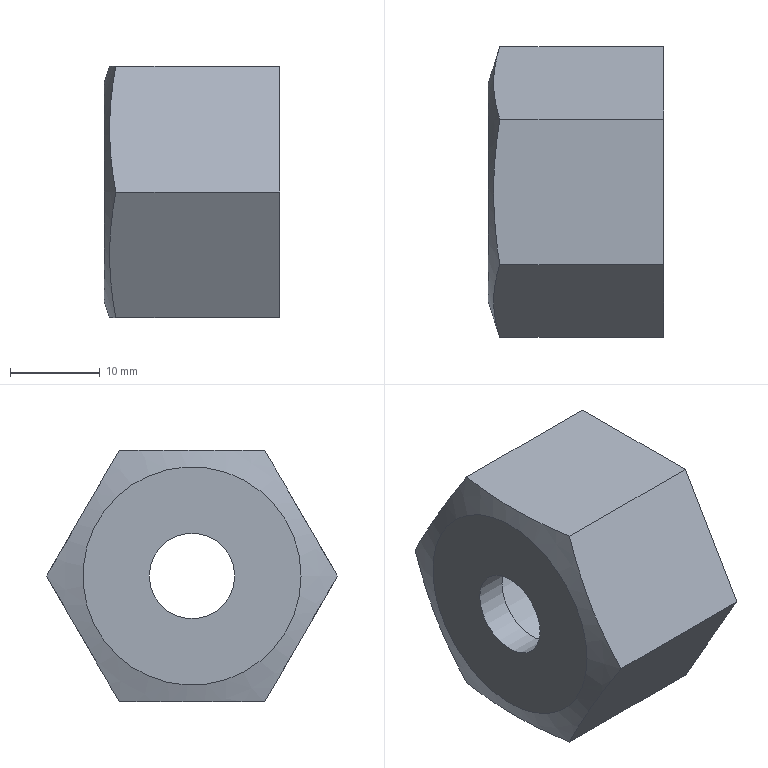Component | NX | LARGE_NUT | 1 solid | 12 faces | box 19.5 x 32.33 x 28 mm | volume 5656 mm3 | plane 9 | cylinder 2 | cone 1 | commonest cylinder face diameters 24 x1 9.5 x1
STEP:
#1=CARTESIAN_POINT('',(0.,0.,0.));
#2=DIRECTION('',(0.,0.,1.));
#3=DIRECTION('',(1.,0.,0.));
#4=AXIS2_PLACEMENT_3D('',#1,#2,#3);
#5=CARTESIAN_POINT('',(-168.222,-8.083,269.5));
#6=VERTEX_POINT('',#5);
#7=CARTESIAN_POINT('',(-150.,-8.083,269.5));
#8=VERTEX_POINT('',#7);
#9=CARTESIAN_POINT('',(-169.5,-8.083,269.5));
#10=DIRECTION('',(1.,0.,0.));
#11=VECTOR('',#10,1.);
#12=LINE('',#9,#11);
#13=CARTESIAN_POINT('',(-169.5,-16.166,255.5));
#14=DIRECTION('',(0.,0.866,-0.5));
#15=DIRECTION('',(0.,-0.5,-0.866));
#16=AXIS2_PLACEMENT_3D('',#13,#14,#15);
#17=PLANE('',#16);
#18=CARTESIAN_POINT('',(-16.166,0.));
#19=DIRECTION('',(0.,-1.));
#20=VECTOR('',#19,1.);
#21=LINE('',#18,#20);
#22=(GEOMETRIC_REPRESENTATION_CONTEXT(2)PARAMETRIC_REPRESENTATION_CONTEXT()REPRESENTATION_CONTEXT('',''));
#23=DEFINITIONAL_REPRESENTATION('',(#21),#22);
#24=PCURVE('',#17,#23);
#25=CARTESIAN_POINT('',(-169.5,-8.083,269.5));
#26=DIRECTION('',(0.,0.,-1.));
#27=DIRECTION('',(0.,-1.,-0.));
#28=AXIS2_PLACEMENT_3D('',#25,#26,#27);
#29=PLANE('',#28);
#30=CARTESIAN_POINT('',(0.,0.));
#31=DIRECTION('',(0.,-1.));
#32=VECTOR('',#31,1.);
#33=LINE('',#30,#32);
#34=(GEOMETRIC_REPRESENTATION_CONTEXT(2)PARAMETRIC_REPRESENTATION_CONTEXT()REPRESENTATION_CONTEXT('',''));
#35=DEFINITIONAL_REPRESENTATION('',(#33),#34);
#36=PCURVE('',#29,#35);
#37=SURFACE_CURVE('',#12,(#24,#36),.PCURVE_S1.);
#38=EDGE_CURVE('',#6,#8,#37,.T.);
#39=ORIENTED_EDGE('',*,*,#38,.F.);
#40=CARTESIAN_POINT('',(-168.222,-16.166,255.5));
#41=VERTEX_POINT('',#40);
#42=CARTESIAN_POINT('',(-168.222,-8.083,269.5));
#43=CARTESIAN_POINT('',(-168.648,-9.43,267.167));
#44=CARTESIAN_POINT('',(-169.166,-12.124,262.5));
#45=CARTESIAN_POINT('',(-168.648,-14.819,257.833));
#46=CARTESIAN_POINT('',(-168.222,-16.166,255.5));
#47=B_SPLINE_CURVE_WITH_KNOTS('',3,(#42,#43,#44,#45,#46),.UNSPECIFIED.,.F.,.F.,(4,1,4),(0.,0.5,1.),.QUASI_UNIFORM_KNOTS.);
#48=CARTESIAN_POINT('',(-16.166,-1.278));
#49=CARTESIAN_POINT('',(-13.472,-0.8519));
#50=CARTESIAN_POINT('',(-8.083,-0.3342));
#51=CARTESIAN_POINT('',(-2.694,-0.8519));
#52=CARTESIAN_POINT('',(0.,-1.278));
#53=B_SPLINE_CURVE_WITH_KNOTS('',3,(#48,#49,#50,#51,#52),.UNSPECIFIED.,.F.,.F.,(4,1,4),(0.,0.5,1.),.QUASI_UNIFORM_KNOTS.);
#54=(GEOMETRIC_REPRESENTATION_CONTEXT(2)PARAMETRIC_REPRESENTATION_CONTEXT()REPRESENTATION_CONTEXT('',''));
#55=DEFINITIONAL_REPRESENTATION('',(#53),#54);
#56=PCURVE('',#17,#55);
#57=CARTESIAN_POINT('',(-169.5,-0.,255.5));
#58=DIRECTION('',(1.,0.,0.));
#59=DIRECTION('',(0.,-1.,0.));
#60=AXIS2_PLACEMENT_3D('',#57,#58,#59);
#61=CONICAL_SURFACE('',#60,12.124,1.265);
#62=CARTESIAN_POINT('',(5.236,1.278));
#63=CARTESIAN_POINT('',(5.249,1.239));
#64=CARTESIAN_POINT('',(5.276,1.164));
#65=CARTESIAN_POINT('',(5.318,1.061));
#66=CARTESIAN_POINT('',(5.362,0.966));
#67=CARTESIAN_POINT('',(5.407,0.8809));
#68=CARTESIAN_POINT('',(5.454,0.8058));
#69=CARTESIAN_POINT('',(5.503,0.7413));
#70=CARTESIAN_POINT('',(5.552,0.6878));
#71=CARTESIAN_POINT('',(5.603,0.6458));
#72=CARTESIAN_POINT('',(5.655,0.6155));
#73=CARTESIAN_POINT('',(5.707,0.5972));
#74=CARTESIAN_POINT('',(5.76,0.591));
#75=CARTESIAN_POINT('',(5.812,0.5972));
#76=CARTESIAN_POINT('',(5.864,0.6155));
#77=CARTESIAN_POINT('',(5.916,0.6458));
#78=CARTESIAN_POINT('',(5.967,0.6878));
#79=CARTESIAN_POINT('',(6.016,0.7413));
#80=CARTESIAN_POINT('',(6.065,0.8058));
#81=CARTESIAN_POINT('',(6.112,0.8809));
#82=CARTESIAN_POINT('',(6.157,0.966));
#83=CARTESIAN_POINT('',(6.201,1.061));
#84=CARTESIAN_POINT('',(6.243,1.164));
#85=CARTESIAN_POINT('',(6.27,1.239));
#86=CARTESIAN_POINT('',(6.283,1.278));
#87=B_SPLINE_CURVE_WITH_KNOTS('',3,(#62,#63,#64,#65,#66,#67,#68,#69,#70,#71,#72,#73,#74,#75,#76,#77,#78,#79,#80,#81,#82,#83,#84,#85,#86),.UNSPECIFIED.,.F.,.F.,(4,1,1,1,1,1,1,1,1,1,1,1,1,1,1,1,1,1,1,1,1,1,4),(0.,0.04545,0.09091,0.1364,0.1818,0.2273,0.2727,0.3182,0.3636,0.4091,0.4545,0.5,0.5455,0.5909,0.6364,0.6818,0.7273,0.7727,0.8182,0.8636,0.9091,0.9545,1.),.QUASI_UNIFORM_KNOTS.);
#88=(GEOMETRIC_REPRESENTATION_CONTEXT(2)PARAMETRIC_REPRESENTATION_CONTEXT()REPRESENTATION_CONTEXT('',''));
#89=DEFINITIONAL_REPRESENTATION('',(#87),#88);
#90=PCURVE('',#61,#89);
#91=SURFACE_CURVE('',#47,(#56,#90),.PCURVE_S1.);
#92=EDGE_CURVE('',#6,#41,#91,.T.);
#93=ORIENTED_EDGE('',*,*,#92,.T.);
#94=CARTESIAN_POINT('',(-150.,-16.166,255.5));
#95=VERTEX_POINT('',#94);
#96=CARTESIAN_POINT('',(-169.5,-16.166,255.5));
#97=DIRECTION('',(1.,0.,0.));
#98=VECTOR('',#97,1.);
#99=LINE('',#96,#98);
#100=CARTESIAN_POINT('',(0.,0.));
#101=DIRECTION('',(0.,-1.));
#102=VECTOR('',#101,1.);
#103=LINE('',#100,#102);
#104=(GEOMETRIC_REPRESENTATION_CONTEXT(2)PARAMETRIC_REPRESENTATION_CONTEXT()REPRESENTATION_CONTEXT('',''));
#105=DEFINITIONAL_REPRESENTATION('',(#103),#104);
#106=PCURVE('',#17,#105);
#107=CARTESIAN_POINT('',(-169.5,-8.083,241.5));
#108=DIRECTION('',(0.,0.866,0.5));
#109=DIRECTION('',(0.,0.5,-0.866));
#110=AXIS2_PLACEMENT_3D('',#107,#108,#109);
#111=PLANE('',#110);
#112=CARTESIAN_POINT('',(-16.166,0.));
#113=DIRECTION('',(0.,-1.));
#114=VECTOR('',#113,1.);
#115=LINE('',#112,#114);
#116=(GEOMETRIC_REPRESENTATION_CONTEXT(2)PARAMETRIC_REPRESENTATION_CONTEXT()REPRESENTATION_CONTEXT('',''));
#117=DEFINITIONAL_REPRESENTATION('',(#115),#116);
#118=PCURVE('',#111,#117);
#119=SURFACE_CURVE('',#99,(#106,#118),.PCURVE_S1.);
#120=EDGE_CURVE('',#41,#95,#119,.T.);
#121=ORIENTED_EDGE('',*,*,#120,.T.);
#122=CARTESIAN_POINT('',(-150.,-16.166,255.5));
#123=DIRECTION('',(0.,0.5,0.866));
#124=VECTOR('',#123,1.);
#125=LINE('',#122,#124);
#126=CARTESIAN_POINT('',(0.,-19.5));
#127=DIRECTION('',(-1.,0.));
#128=VECTOR('',#127,1.);
#129=LINE('',#126,#128);
#130=(GEOMETRIC_REPRESENTATION_CONTEXT(2)PARAMETRIC_REPRESENTATION_CONTEXT()REPRESENTATION_CONTEXT('',''));
#131=DEFINITIONAL_REPRESENTATION('',(#129),#130);
#132=PCURVE('',#17,#131);
#133=CARTESIAN_POINT('',(-150.,-0.,255.5));
#134=DIRECTION('',(-1.,0.,0.));
#135=DIRECTION('',(0.,1.,0.));
#136=AXIS2_PLACEMENT_3D('',#133,#134,#135);
#137=PLANE('',#136);
#138=CARTESIAN_POINT('',(-16.166,0.));
#139=DIRECTION('',(0.5,-0.866));
#140=VECTOR('',#139,1.);
#141=LINE('',#138,#140);
#142=(GEOMETRIC_REPRESENTATION_CONTEXT(2)PARAMETRIC_REPRESENTATION_CONTEXT()REPRESENTATION_CONTEXT('',''));
#143=DEFINITIONAL_REPRESENTATION('',(#141),#142);
#144=PCURVE('',#137,#143);
#145=SURFACE_CURVE('',#125,(#132,#144),.PCURVE_S1.);
#146=EDGE_CURVE('',#95,#8,#145,.T.);
#147=ORIENTED_EDGE('',*,*,#146,.T.);
#148=EDGE_LOOP('',(#39,#93,#121,#147));
#149=FACE_BOUND('',#148,.T.);
#150=ADVANCED_FACE('',(#149),#17,.F.);
#151=CARTESIAN_POINT('',(-168.222,8.083,269.5));
#152=VERTEX_POINT('',#151);
#153=CARTESIAN_POINT('',(-150.,8.083,269.5));
#154=VERTEX_POINT('',#153);
#155=CARTESIAN_POINT('',(-169.5,8.083,269.5));
#156=DIRECTION('',(1.,0.,0.));
#157=VECTOR('',#156,1.);
#158=LINE('',#155,#157);
#159=CARTESIAN_POINT('',(-16.166,0.));
#160=DIRECTION('',(0.,-1.));
#161=VECTOR('',#160,1.);
#162=LINE('',#159,#161);
#163=(GEOMETRIC_REPRESENTATION_CONTEXT(2)PARAMETRIC_REPRESENTATION_CONTEXT()REPRESENTATION_CONTEXT('',''));
#164=DEFINITIONAL_REPRESENTATION('',(#162),#163);
#165=PCURVE('',#29,#164);
#166=CARTESIAN_POINT('',(-169.5,8.083,269.5));
#167=DIRECTION('',(0.,-0.866,-0.5));
#168=DIRECTION('',(0.,-0.5,0.866));
#169=AXIS2_PLACEMENT_3D('',#166,#167,#168);
#170=PLANE('',#169);
#171=CARTESIAN_POINT('',(0.,0.));
#172=DIRECTION('',(0.,-1.));
#173=VECTOR('',#172,1.);
#174=LINE('',#171,#173);
#175=(GEOMETRIC_REPRESENTATION_CONTEXT(2)PARAMETRIC_REPRESENTATION_CONTEXT()REPRESENTATION_CONTEXT('',''));
#176=DEFINITIONAL_REPRESENTATION('',(#174),#175);
#177=PCURVE('',#170,#176);
#178=SURFACE_CURVE('',#158,(#165,#177),.PCURVE_S1.);
#179=EDGE_CURVE('',#152,#154,#178,.T.);
#180=ORIENTED_EDGE('',*,*,#179,.F.);
#181=CARTESIAN_POINT('',(-168.222,8.083,269.5));
#182=CARTESIAN_POINT('',(-168.646,5.403,269.5));
#183=CARTESIAN_POINT('',(-168.906,2.717,269.5));
#184=CARTESIAN_POINT('',(-168.908,-2.675,269.5));
#185=CARTESIAN_POINT('',(-168.647,-5.393,269.5));
#186=CARTESIAN_POINT('',(-168.222,-8.083,269.5));
#187=B_SPLINE_CURVE_WITH_KNOTS('',3,(#181,#182,#183,#184,#185,#186),.UNSPECIFIED.,.F.,.F.,(4,2,4),(0.,0.5,1.),.UNSPECIFIED.);
#188=CARTESIAN_POINT('',(-16.166,-1.278));
#189=CARTESIAN_POINT('',(-13.486,-0.8542));
#190=CARTESIAN_POINT('',(-10.799,-0.5944));
#191=CARTESIAN_POINT('',(-5.408,-0.5918));
#192=CARTESIAN_POINT('',(-2.69,-0.8527));
#193=CARTESIAN_POINT('',(0.,-1.278));
#194=B_SPLINE_CURVE_WITH_KNOTS('',3,(#188,#189,#190,#191,#192,#193),.UNSPECIFIED.,.F.,.F.,(4,2,4),(0.,0.5,1.),.UNSPECIFIED.);
#195=(GEOMETRIC_REPRESENTATION_CONTEXT(2)PARAMETRIC_REPRESENTATION_CONTEXT()REPRESENTATION_CONTEXT('',''));
#196=DEFINITIONAL_REPRESENTATION('',(#194),#195);
#197=PCURVE('',#29,#196);
#198=CARTESIAN_POINT('',(4.189,1.278));
#199=CARTESIAN_POINT('',(4.202,1.239));
#200=CARTESIAN_POINT('',(4.229,1.165));
#201=CARTESIAN_POINT('',(4.27,1.062));
#202=CARTESIAN_POINT('',(4.314,0.9673));
#203=CARTESIAN_POINT('',(4.359,0.8823));
#204=CARTESIAN_POINT('',(4.406,0.8073));
#205=CARTESIAN_POINT('',(4.454,0.7427));
#206=CARTESIAN_POINT('',(4.504,0.6891));
#207=CARTESIAN_POINT('',(4.555,0.6468));
#208=CARTESIAN_POINT('',(4.606,0.6162));
#209=CARTESIAN_POINT('',(4.658,0.5975));
#210=CARTESIAN_POINT('',(4.711,0.591));
#211=CARTESIAN_POINT('',(4.763,0.5968));
#212=CARTESIAN_POINT('',(4.816,0.6149));
#213=CARTESIAN_POINT('',(4.868,0.645));
#214=CARTESIAN_POINT('',(4.919,0.687));
#215=CARTESIAN_POINT('',(4.969,0.7406));
#216=CARTESIAN_POINT('',(5.017,0.8052));
#217=CARTESIAN_POINT('',(5.065,0.8805));
#218=CARTESIAN_POINT('',(5.11,0.9658));
#219=CARTESIAN_POINT('',(5.154,1.061));
#220=CARTESIAN_POINT('',(5.196,1.165));
#221=CARTESIAN_POINT('',(5.223,1.239));
#222=CARTESIAN_POINT('',(5.236,1.278));
#223=B_SPLINE_CURVE_WITH_KNOTS('',3,(#198,#199,#200,#201,#202,#203,#204,#205,#206,#207,#208,#209,#210,#211,#212,#213,#214,#215,#216,#217,#218,#219,#220,#221,#222),.UNSPECIFIED.,.F.,.F.,(4,1,1,1,1,1,1,1,1,1,1,1,1,1,1,1,1,1,1,1,1,1,4),(0.,0.04545,0.09091,0.1364,0.1818,0.2273,0.2727,0.3182,0.3636,0.4091,0.4545,0.5,0.5455,0.5909,0.6364,0.6818,0.7273,0.7727,0.8182,0.8636,0.9091,0.9545,1.),.QUASI_UNIFORM_KNOTS.);
#224=(GEOMETRIC_REPRESENTATION_CONTEXT(2)PARAMETRIC_REPRESENTATION_CONTEXT()REPRESENTATION_CONTEXT('',''));
#225=DEFINITIONAL_REPRESENTATION('',(#223),#224);
#226=PCURVE('',#61,#225);
#227=SURFACE_CURVE('',#187,(#197,#226),.PCURVE_S1.);
#228=EDGE_CURVE('',#152,#6,#227,.T.);
#229=ORIENTED_EDGE('',*,*,#228,.T.);
#230=ORIENTED_EDGE('',*,*,#38,.T.);
#231=CARTESIAN_POINT('',(-150.,-8.083,269.5));
#232=DIRECTION('',(0.,1.,0.));
#233=VECTOR('',#232,1.);
#234=LINE('',#231,#233);
#235=CARTESIAN_POINT('',(0.,-19.5));
#236=DIRECTION('',(-1.,0.));
#237=VECTOR('',#236,1.);
#238=LINE('',#235,#237);
#239=(GEOMETRIC_REPRESENTATION_CONTEXT(2)PARAMETRIC_REPRESENTATION_CONTEXT()REPRESENTATION_CONTEXT('',''));
#240=DEFINITIONAL_REPRESENTATION('',(#238),#239);
#241=PCURVE('',#29,#240);
#242=CARTESIAN_POINT('',(-8.083,-14.));
#243=DIRECTION('',(1.,-0.));
#244=VECTOR('',#243,1.);
#245=LINE('',#242,#244);
#246=(GEOMETRIC_REPRESENTATION_CONTEXT(2)PARAMETRIC_REPRESENTATION_CONTEXT()REPRESENTATION_CONTEXT('',''));
#247=DEFINITIONAL_REPRESENTATION('',(#245),#246);
#248=PCURVE('',#137,#247);
#249=SURFACE_CURVE('',#234,(#241,#248),.PCURVE_S1.);
#250=EDGE_CURVE('',#8,#154,#249,.T.);
#251=ORIENTED_EDGE('',*,*,#250,.T.);
#252=EDGE_LOOP('',(#180,#229,#230,#251));
#253=FACE_BOUND('',#252,.T.);
#254=ADVANCED_FACE('',(#253),#29,.F.);
#255=CARTESIAN_POINT('',(-168.222,16.166,255.5));
#256=VERTEX_POINT('',#255);
#257=CARTESIAN_POINT('',(-150.,16.166,255.5));
#258=VERTEX_POINT('',#257);
#259=CARTESIAN_POINT('',(-169.5,16.166,255.5));
#260=DIRECTION('',(1.,0.,0.));
#261=VECTOR('',#260,1.);
#262=LINE('',#259,#261);
#263=CARTESIAN_POINT('',(-16.166,0.));
#264=DIRECTION('',(0.,-1.));
#265=VECTOR('',#264,1.);
#266=LINE('',#263,#265);
#267=(GEOMETRIC_REPRESENTATION_CONTEXT(2)PARAMETRIC_REPRESENTATION_CONTEXT()REPRESENTATION_CONTEXT('',''));
#268=DEFINITIONAL_REPRESENTATION('',(#266),#267);
#269=PCURVE('',#170,#268);
#270=CARTESIAN_POINT('',(-169.5,16.166,255.5));
#271=DIRECTION('',(0.,-0.866,0.5));
#272=DIRECTION('',(0.,0.5,0.866));
#273=AXIS2_PLACEMENT_3D('',#270,#271,#272);
#274=PLANE('',#273);
#275=CARTESIAN_POINT('',(0.,0.));
#276=DIRECTION('',(0.,-1.));
#277=VECTOR('',#276,1.);
#278=LINE('',#275,#277);
#279=(GEOMETRIC_REPRESENTATION_CONTEXT(2)PARAMETRIC_REPRESENTATION_CONTEXT()REPRESENTATION_CONTEXT('',''));
#280=DEFINITIONAL_REPRESENTATION('',(#278),#279);
#281=PCURVE('',#274,#280);
#282=SURFACE_CURVE('',#262,(#269,#281),.PCURVE_S1.);
#283=EDGE_CURVE('',#256,#258,#282,.T.);
#284=ORIENTED_EDGE('',*,*,#283,.F.);
#285=CARTESIAN_POINT('',(-168.222,16.166,255.5));
#286=CARTESIAN_POINT('',(-168.648,14.819,257.833));
#287=CARTESIAN_POINT('',(-169.166,12.124,262.5));
#288=CARTESIAN_POINT('',(-168.648,9.43,267.167));
#289=CARTESIAN_POINT('',(-168.222,8.083,269.5));
#290=B_SPLINE_CURVE_WITH_KNOTS('',3,(#285,#286,#287,#288,#289),.UNSPECIFIED.,.F.,.F.,(4,1,4),(0.,0.5,1.),.QUASI_UNIFORM_KNOTS.);
#291=CARTESIAN_POINT('',(-16.166,-1.278));
#292=CARTESIAN_POINT('',(-13.472,-0.8519));
#293=CARTESIAN_POINT('',(-8.083,-0.3342));
#294=CARTESIAN_POINT('',(-2.694,-0.8519));
#295=CARTESIAN_POINT('',(0.,-1.278));
#296=B_SPLINE_CURVE_WITH_KNOTS('',3,(#291,#292,#293,#294,#295),.UNSPECIFIED.,.F.,.F.,(4,1,4),(0.,0.5,1.),.QUASI_UNIFORM_KNOTS.);
#297=(GEOMETRIC_REPRESENTATION_CONTEXT(2)PARAMETRIC_REPRESENTATION_CONTEXT()REPRESENTATION_CONTEXT('',''));
#298=DEFINITIONAL_REPRESENTATION('',(#296),#297);
#299=PCURVE('',#170,#298);
#300=CARTESIAN_POINT('',(3.142,1.278));
#301=CARTESIAN_POINT('',(3.155,1.239));
#302=CARTESIAN_POINT('',(3.182,1.164));
#303=CARTESIAN_POINT('',(3.224,1.061));
#304=CARTESIAN_POINT('',(3.267,0.966));
#305=CARTESIAN_POINT('',(3.313,0.8809));
#306=CARTESIAN_POINT('',(3.36,0.8058));
#307=CARTESIAN_POINT('',(3.408,0.7413));
#308=CARTESIAN_POINT('',(3.458,0.6878));
#309=CARTESIAN_POINT('',(3.509,0.6458));
#310=CARTESIAN_POINT('',(3.561,0.6155));
#311=CARTESIAN_POINT('',(3.613,0.5972));
#312=CARTESIAN_POINT('',(3.665,0.591));
#313=CARTESIAN_POINT('',(3.718,0.5972));
#314=CARTESIAN_POINT('',(3.77,0.6155));
#315=CARTESIAN_POINT('',(3.822,0.6458));
#316=CARTESIAN_POINT('',(3.872,0.6878));
#317=CARTESIAN_POINT('',(3.922,0.7413));
#318=CARTESIAN_POINT('',(3.971,0.8058));
#319=CARTESIAN_POINT('',(4.018,0.8809));
#320=CARTESIAN_POINT('',(4.063,0.966));
#321=CARTESIAN_POINT('',(4.107,1.061));
#322=CARTESIAN_POINT('',(4.149,1.164));
#323=CARTESIAN_POINT('',(4.176,1.239));
#324=CARTESIAN_POINT('',(4.189,1.278));
#325=B_SPLINE_CURVE_WITH_KNOTS('',3,(#300,#301,#302,#303,#304,#305,#306,#307,#308,#309,#310,#311,#312,#313,#314,#315,#316,#317,#318,#319,#320,#321,#322,#323,#324),.UNSPECIFIED.,.F.,.F.,(4,1,1,1,1,1,1,1,1,1,1,1,1,1,1,1,1,1,1,1,1,1,4),(0.,0.04545,0.09091,0.1364,0.1818,0.2273,0.2727,0.3182,0.3636,0.4091,0.4545,0.5,0.5455,0.5909,0.6364,0.6818,0.7273,0.7727,0.8182,0.8636,0.9091,0.9545,1.),.QUASI_UNIFORM_KNOTS.);
#326=(GEOMETRIC_REPRESENTATION_CONTEXT(2)PARAMETRIC_REPRESENTATION_CONTEXT()REPRESENTATION_CONTEXT('',''));
#327=DEFINITIONAL_REPRESENTATION('',(#325),#326);
#328=PCURVE('',#61,#327);
#329=SURFACE_CURVE('',#290,(#299,#328),.PCURVE_S1.);
#330=EDGE_CURVE('',#256,#152,#329,.T.);
#331=ORIENTED_EDGE('',*,*,#330,.T.);
#332=ORIENTED_EDGE('',*,*,#179,.T.);
#333=CARTESIAN_POINT('',(-150.,8.083,269.5));
#334=DIRECTION('',(0.,0.5,-0.866));
#335=VECTOR('',#334,1.);
#336=LINE('',#333,#335);
#337=CARTESIAN_POINT('',(0.,-19.5));
#338=DIRECTION('',(-1.,0.));
#339=VECTOR('',#338,1.);
#340=LINE('',#337,#339);
#341=(GEOMETRIC_REPRESENTATION_CONTEXT(2)PARAMETRIC_REPRESENTATION_CONTEXT()REPRESENTATION_CONTEXT('',''));
#342=DEFINITIONAL_REPRESENTATION('',(#340),#341);
#343=PCURVE('',#170,#342);
#344=CARTESIAN_POINT('',(8.083,-14.));
#345=DIRECTION('',(0.5,0.866));
#346=VECTOR('',#345,1.);
#347=LINE('',#344,#346);
#348=(GEOMETRIC_REPRESENTATION_CONTEXT(2)PARAMETRIC_REPRESENTATION_CONTEXT()REPRESENTATION_CONTEXT('',''));
#349=DEFINITIONAL_REPRESENTATION('',(#347),#348);
#350=PCURVE('',#137,#349);
#351=SURFACE_CURVE('',#336,(#343,#350),.PCURVE_S1.);
#352=EDGE_CURVE('',#154,#258,#351,.T.);
#353=ORIENTED_EDGE('',*,*,#352,.T.);
#354=EDGE_LOOP('',(#284,#331,#332,#353));
#355=FACE_BOUND('',#354,.T.);
#356=ADVANCED_FACE('',(#355),#170,.F.);
#357=CARTESIAN_POINT('',(-168.222,8.083,241.5));
#358=VERTEX_POINT('',#357);
#359=CARTESIAN_POINT('',(-150.,8.083,241.5));
#360=VERTEX_POINT('',#359);
#361=CARTESIAN_POINT('',(-169.5,8.083,241.5));
#362=DIRECTION('',(1.,0.,0.));
#363=VECTOR('',#362,1.);
#364=LINE('',#361,#363);
#365=CARTESIAN_POINT('',(-16.166,0.));
#366=DIRECTION('',(0.,-1.));
#367=VECTOR('',#366,1.);
#368=LINE('',#365,#367);
#369=(GEOMETRIC_REPRESENTATION_CONTEXT(2)PARAMETRIC_REPRESENTATION_CONTEXT()REPRESENTATION_CONTEXT('',''));
#370=DEFINITIONAL_REPRESENTATION('',(#368),#369);
#371=PCURVE('',#274,#370);
#372=CARTESIAN_POINT('',(-169.5,8.083,241.5));
#373=DIRECTION('',(0.,-0.,1.));
#374=DIRECTION('',(0.,1.,0.));
#375=AXIS2_PLACEMENT_3D('',#372,#373,#374);
#376=PLANE('',#375);
#377=CARTESIAN_POINT('',(0.,0.));
#378=DIRECTION('',(0.,-1.));
#379=VECTOR('',#378,1.);
#380=LINE('',#377,#379);
#381=(GEOMETRIC_REPRESENTATION_CONTEXT(2)PARAMETRIC_REPRESENTATION_CONTEXT()REPRESENTATION_CONTEXT('',''));
#382=DEFINITIONAL_REPRESENTATION('',(#380),#381);
#383=PCURVE('',#376,#382);
#384=SURFACE_CURVE('',#364,(#371,#383),.PCURVE_S1.);
#385=EDGE_CURVE('',#358,#360,#384,.T.);
#386=ORIENTED_EDGE('',*,*,#385,.F.);
#387=CARTESIAN_POINT('',(-168.222,8.083,241.5));
#388=CARTESIAN_POINT('',(-168.648,9.43,243.833));
#389=CARTESIAN_POINT('',(-169.166,12.124,248.5));
#390=CARTESIAN_POINT('',(-168.648,14.819,253.167));
#391=CARTESIAN_POINT('',(-168.222,16.166,255.5));
#392=B_SPLINE_CURVE_WITH_KNOTS('',3,(#387,#388,#389,#390,#391),.UNSPECIFIED.,.F.,.F.,(4,1,4),(0.,0.5,1.),.UNSPECIFIED.);
#393=CARTESIAN_POINT('',(-16.166,-1.278));
#394=CARTESIAN_POINT('',(-13.472,-0.8519));
#395=CARTESIAN_POINT('',(-8.083,-0.3342));
#396=CARTESIAN_POINT('',(-2.694,-0.8519));
#397=CARTESIAN_POINT('',(0.,-1.278));
#398=B_SPLINE_CURVE_WITH_KNOTS('',3,(#393,#394,#395,#396,#397),.UNSPECIFIED.,.F.,.F.,(4,1,4),(0.,0.5,1.),.UNSPECIFIED.);
#399=(GEOMETRIC_REPRESENTATION_CONTEXT(2)PARAMETRIC_REPRESENTATION_CONTEXT()REPRESENTATION_CONTEXT('',''));
#400=DEFINITIONAL_REPRESENTATION('',(#398),#399);
#401=PCURVE('',#274,#400);
#402=CARTESIAN_POINT('',(2.094,1.278));
#403=CARTESIAN_POINT('',(2.108,1.239));
#404=CARTESIAN_POINT('',(2.134,1.164));
#405=CARTESIAN_POINT('',(2.176,1.061));
#406=CARTESIAN_POINT('',(2.22,0.966));
#407=CARTESIAN_POINT('',(2.266,0.8809));
#408=CARTESIAN_POINT('',(2.313,0.8058));
#409=CARTESIAN_POINT('',(2.361,0.7413));
#410=CARTESIAN_POINT('',(2.411,0.6878));
#411=CARTESIAN_POINT('',(2.462,0.6458));
#412=CARTESIAN_POINT('',(2.513,0.6155));
#413=CARTESIAN_POINT('',(2.566,0.5972));
#414=CARTESIAN_POINT('',(2.618,0.591));
#415=CARTESIAN_POINT('',(2.67,0.5972));
#416=CARTESIAN_POINT('',(2.723,0.6155));
#417=CARTESIAN_POINT('',(2.774,0.6458));
#418=CARTESIAN_POINT('',(2.825,0.6878));
#419=CARTESIAN_POINT('',(2.875,0.7413));
#420=CARTESIAN_POINT('',(2.923,0.8058));
#421=CARTESIAN_POINT('',(2.97,0.8809));
#422=CARTESIAN_POINT('',(3.016,0.966));
#423=CARTESIAN_POINT('',(3.06,1.061));
#424=CARTESIAN_POINT('',(3.102,1.164));
#425=CARTESIAN_POINT('',(3.128,1.239));
#426=CARTESIAN_POINT('',(3.142,1.278));
#427=B_SPLINE_CURVE_WITH_KNOTS('',3,(#402,#403,#404,#405,#406,#407,#408,#409,#410,#411,#412,#413,#414,#415,#416,#417,#418,#419,#420,#421,#422,#423,#424,#425,#426),.UNSPECIFIED.,.F.,.F.,(4,1,1,1,1,1,1,1,1,1,1,1,1,1,1,1,1,1,1,1,1,1,4),(0.,0.04545,0.09091,0.1364,0.1818,0.2273,0.2727,0.3182,0.3636,0.4091,0.4545,0.5,0.5455,0.5909,0.6364,0.6818,0.7273,0.7727,0.8182,0.8636,0.9091,0.9545,1.),.QUASI_UNIFORM_KNOTS.);
#428=(GEOMETRIC_REPRESENTATION_CONTEXT(2)PARAMETRIC_REPRESENTATION_CONTEXT()REPRESENTATION_CONTEXT('',''));
#429=DEFINITIONAL_REPRESENTATION('',(#427),#428);
#430=PCURVE('',#61,#429);
#431=SURFACE_CURVE('',#392,(#401,#430),.PCURVE_S1.);
#432=EDGE_CURVE('',#358,#256,#431,.T.);
#433=ORIENTED_EDGE('',*,*,#432,.T.);
#434=ORIENTED_EDGE('',*,*,#283,.T.);
#435=CARTESIAN_POINT('',(-150.,16.166,255.5));
#436=DIRECTION('',(0.,-0.5,-0.866));
#437=VECTOR('',#436,1.);
#438=LINE('',#435,#437);
#439=CARTESIAN_POINT('',(0.,-19.5));
#440=DIRECTION('',(-1.,0.));
#441=VECTOR('',#440,1.);
#442=LINE('',#439,#441);
#443=(GEOMETRIC_REPRESENTATION_CONTEXT(2)PARAMETRIC_REPRESENTATION_CONTEXT()REPRESENTATION_CONTEXT('',''));
#444=DEFINITIONAL_REPRESENTATION('',(#442),#443);
#445=PCURVE('',#274,#444);
#446=CARTESIAN_POINT('',(16.166,0.));
#447=DIRECTION('',(-0.5,0.866));
#448=VECTOR('',#447,1.);
#449=LINE('',#446,#448);
#450=(GEOMETRIC_REPRESENTATION_CONTEXT(2)PARAMETRIC_REPRESENTATION_CONTEXT()REPRESENTATION_CONTEXT('',''));
#451=DEFINITIONAL_REPRESENTATION('',(#449),#450);
#452=PCURVE('',#137,#451);
#453=SURFACE_CURVE('',#438,(#445,#452),.PCURVE_S1.);
#454=EDGE_CURVE('',#258,#360,#453,.T.);
#455=ORIENTED_EDGE('',*,*,#454,.T.);
#456=EDGE_LOOP('',(#386,#433,#434,#455));
#457=FACE_BOUND('',#456,.T.);
#458=ADVANCED_FACE('',(#457),#274,.F.);
#459=CARTESIAN_POINT('',(-168.222,-8.083,241.5));
#460=VERTEX_POINT('',#459);
#461=CARTESIAN_POINT('',(-150.,-8.083,241.5));
#462=VERTEX_POINT('',#461);
#463=CARTESIAN_POINT('',(-169.5,-8.083,241.5));
#464=DIRECTION('',(1.,0.,0.));
#465=VECTOR('',#464,1.);
#466=LINE('',#463,#465);
#467=CARTESIAN_POINT('',(-16.166,0.));
#468=DIRECTION('',(0.,-1.));
#469=VECTOR('',#468,1.);
#470=LINE('',#467,#469);
#471=(GEOMETRIC_REPRESENTATION_CONTEXT(2)PARAMETRIC_REPRESENTATION_CONTEXT()REPRESENTATION_CONTEXT('',''));
#472=DEFINITIONAL_REPRESENTATION('',(#470),#471);
#473=PCURVE('',#376,#472);
#474=CARTESIAN_POINT('',(0.,0.));
#475=DIRECTION('',(0.,-1.));
#476=VECTOR('',#475,1.);
#477=LINE('',#474,#476);
#478=(GEOMETRIC_REPRESENTATION_CONTEXT(2)PARAMETRIC_REPRESENTATION_CONTEXT()REPRESENTATION_CONTEXT('',''));
#479=DEFINITIONAL_REPRESENTATION('',(#477),#478);
#480=PCURVE('',#111,#479);
#481=SURFACE_CURVE('',#466,(#473,#480),.PCURVE_S1.);
#482=EDGE_CURVE('',#460,#462,#481,.T.);
#483=ORIENTED_EDGE('',*,*,#482,.F.);
#484=CARTESIAN_POINT('',(-168.222,-8.083,241.5));
#485=CARTESIAN_POINT('',(-168.647,-5.393,241.5));
#486=CARTESIAN_POINT('',(-168.908,-2.675,241.5));
#487=CARTESIAN_POINT('',(-168.906,2.717,241.5));
#488=CARTESIAN_POINT('',(-168.646,5.403,241.5));
#489=CARTESIAN_POINT('',(-168.222,8.083,241.5));
#490=B_SPLINE_CURVE_WITH_KNOTS('',3,(#484,#485,#486,#487,#488,#489),.UNSPECIFIED.,.F.,.F.,(4,2,4),(0.,0.5,1.),.UNSPECIFIED.);
#491=CARTESIAN_POINT('',(-16.166,-1.278));
#492=CARTESIAN_POINT('',(-13.476,-0.8527));
#493=CARTESIAN_POINT('',(-10.758,-0.5918));
#494=CARTESIAN_POINT('',(-5.366,-0.5944));
#495=CARTESIAN_POINT('',(-2.68,-0.8542));
#496=CARTESIAN_POINT('',(0.,-1.278));
#497=B_SPLINE_CURVE_WITH_KNOTS('',3,(#491,#492,#493,#494,#495,#496),.UNSPECIFIED.,.F.,.F.,(4,2,4),(0.,0.5,1.),.UNSPECIFIED.);
#498=(GEOMETRIC_REPRESENTATION_CONTEXT(2)PARAMETRIC_REPRESENTATION_CONTEXT()REPRESENTATION_CONTEXT('',''));
#499=DEFINITIONAL_REPRESENTATION('',(#497),#498);
#500=PCURVE('',#376,#499);
#501=CARTESIAN_POINT('',(1.047,1.278));
#502=CARTESIAN_POINT('',(1.06,1.239));
#503=CARTESIAN_POINT('',(1.087,1.165));
#504=CARTESIAN_POINT('',(1.129,1.061));
#505=CARTESIAN_POINT('',(1.173,0.9658));
#506=CARTESIAN_POINT('',(1.219,0.8805));
#507=CARTESIAN_POINT('',(1.266,0.8052));
#508=CARTESIAN_POINT('',(1.315,0.7406));
#509=CARTESIAN_POINT('',(1.365,0.687));
#510=CARTESIAN_POINT('',(1.416,0.645));
#511=CARTESIAN_POINT('',(1.467,0.6149));
#512=CARTESIAN_POINT('',(1.52,0.5968));
#513=CARTESIAN_POINT('',(1.572,0.591));
#514=CARTESIAN_POINT('',(1.625,0.5975));
#515=CARTESIAN_POINT('',(1.677,0.6162));
#516=CARTESIAN_POINT('',(1.729,0.6468));
#517=CARTESIAN_POINT('',(1.779,0.6891));
#518=CARTESIAN_POINT('',(1.829,0.7427));
#519=CARTESIAN_POINT('',(1.877,0.8073));
#520=CARTESIAN_POINT('',(1.924,0.8823));
#521=CARTESIAN_POINT('',(1.969,0.9673));
#522=CARTESIAN_POINT('',(2.013,1.062));
#523=CARTESIAN_POINT('',(2.055,1.165));
#524=CARTESIAN_POINT('',(2.081,1.239));
#525=CARTESIAN_POINT('',(2.094,1.278));
#526=B_SPLINE_CURVE_WITH_KNOTS('',3,(#501,#502,#503,#504,#505,#506,#507,#508,#509,#510,#511,#512,#513,#514,#515,#516,#517,#518,#519,#520,#521,#522,#523,#524,#525),.UNSPECIFIED.,.F.,.F.,(4,1,1,1,1,1,1,1,1,1,1,1,1,1,1,1,1,1,1,1,1,1,4),(0.,0.04545,0.09091,0.1364,0.1818,0.2273,0.2727,0.3182,0.3636,0.4091,0.4545,0.5,0.5455,0.5909,0.6364,0.6818,0.7273,0.7727,0.8182,0.8636,0.9091,0.9545,1.),.QUASI_UNIFORM_KNOTS.);
#527=(GEOMETRIC_REPRESENTATION_CONTEXT(2)PARAMETRIC_REPRESENTATION_CONTEXT()REPRESENTATION_CONTEXT('',''));
#528=DEFINITIONAL_REPRESENTATION('',(#526),#527);
#529=PCURVE('',#61,#528);
#530=SURFACE_CURVE('',#490,(#500,#529),.PCURVE_S1.);
#531=EDGE_CURVE('',#460,#358,#530,.T.);
#532=ORIENTED_EDGE('',*,*,#531,.T.);
#533=ORIENTED_EDGE('',*,*,#385,.T.);
#534=CARTESIAN_POINT('',(-150.,8.083,241.5));
#535=DIRECTION('',(0.,-1.,-0.));
#536=VECTOR('',#535,1.);
#537=LINE('',#534,#536);
#538=CARTESIAN_POINT('',(0.,-19.5));
#539=DIRECTION('',(-1.,0.));
#540=VECTOR('',#539,1.);
#541=LINE('',#538,#540);
#542=(GEOMETRIC_REPRESENTATION_CONTEXT(2)PARAMETRIC_REPRESENTATION_CONTEXT()REPRESENTATION_CONTEXT('',''));
#543=DEFINITIONAL_REPRESENTATION('',(#541),#542);
#544=PCURVE('',#376,#543);
#545=CARTESIAN_POINT('',(8.083,14.));
#546=DIRECTION('',(-1.,0.));
#547=VECTOR('',#546,1.);
#548=LINE('',#545,#547);
#549=(GEOMETRIC_REPRESENTATION_CONTEXT(2)PARAMETRIC_REPRESENTATION_CONTEXT()REPRESENTATION_CONTEXT('',''));
#550=DEFINITIONAL_REPRESENTATION('',(#548),#549);
#551=PCURVE('',#137,#550);
#552=SURFACE_CURVE('',#537,(#544,#551),.PCURVE_S1.);
#553=EDGE_CURVE('',#360,#462,#552,.T.);
#554=ORIENTED_EDGE('',*,*,#553,.T.);
#555=EDGE_LOOP('',(#483,#532,#533,#554));
#556=FACE_BOUND('',#555,.T.);
#557=ADVANCED_FACE('',(#556),#376,.F.);
#558=ORIENTED_EDGE('',*,*,#120,.F.);
#559=CARTESIAN_POINT('',(-168.222,-16.166,255.5));
#560=CARTESIAN_POINT('',(-168.648,-14.819,253.167));
#561=CARTESIAN_POINT('',(-169.166,-12.124,248.5));
#562=CARTESIAN_POINT('',(-168.648,-9.43,243.833));
#563=CARTESIAN_POINT('',(-168.222,-8.083,241.5));
#564=B_SPLINE_CURVE_WITH_KNOTS('',3,(#559,#560,#561,#562,#563),.UNSPECIFIED.,.F.,.F.,(4,1,4),(0.,0.5,1.),.UNSPECIFIED.);
#565=CARTESIAN_POINT('',(-16.166,-1.278));
#566=CARTESIAN_POINT('',(-13.472,-0.8519));
#567=CARTESIAN_POINT('',(-8.083,-0.3342));
#568=CARTESIAN_POINT('',(-2.694,-0.8519));
#569=CARTESIAN_POINT('',(0.,-1.278));
#570=B_SPLINE_CURVE_WITH_KNOTS('',3,(#565,#566,#567,#568,#569),.UNSPECIFIED.,.F.,.F.,(4,1,4),(0.,0.5,1.),.UNSPECIFIED.);
#571=(GEOMETRIC_REPRESENTATION_CONTEXT(2)PARAMETRIC_REPRESENTATION_CONTEXT()REPRESENTATION_CONTEXT('',''));
#572=DEFINITIONAL_REPRESENTATION('',(#570),#571);
#573=PCURVE('',#111,#572);
#574=CARTESIAN_POINT('',(0.,1.278));
#575=CARTESIAN_POINT('',(0.01312,1.239));
#576=CARTESIAN_POINT('',(0.03996,1.164));
#577=CARTESIAN_POINT('',(0.082,1.061));
#578=CARTESIAN_POINT('',(0.1258,0.966));
#579=CARTESIAN_POINT('',(0.1712,0.8809));
#580=CARTESIAN_POINT('',(0.2183,0.8058));
#581=CARTESIAN_POINT('',(0.2667,0.7413));
#582=CARTESIAN_POINT('',(0.3165,0.6878));
#583=CARTESIAN_POINT('',(0.3673,0.6458));
#584=CARTESIAN_POINT('',(0.4189,0.6155));
#585=CARTESIAN_POINT('',(0.4711,0.5972));
#586=CARTESIAN_POINT('',(0.5236,0.591));
#587=CARTESIAN_POINT('',(0.5761,0.5972));
#588=CARTESIAN_POINT('',(0.6283,0.6155));
#589=CARTESIAN_POINT('',(0.6799,0.6458));
#590=CARTESIAN_POINT('',(0.7307,0.6878));
#591=CARTESIAN_POINT('',(0.7805,0.7413));
#592=CARTESIAN_POINT('',(0.8289,0.8058));
#593=CARTESIAN_POINT('',(0.876,0.8809));
#594=CARTESIAN_POINT('',(0.9214,0.966));
#595=CARTESIAN_POINT('',(0.9652,1.061));
#596=CARTESIAN_POINT('',(1.007,1.164));
#597=CARTESIAN_POINT('',(1.034,1.239));
#598=CARTESIAN_POINT('',(1.047,1.278));
#599=B_SPLINE_CURVE_WITH_KNOTS('',3,(#574,#575,#576,#577,#578,#579,#580,#581,#582,#583,#584,#585,#586,#587,#588,#589,#590,#591,#592,#593,#594,#595,#596,#597,#598),.UNSPECIFIED.,.F.,.F.,(4,1,1,1,1,1,1,1,1,1,1,1,1,1,1,1,1,1,1,1,1,1,4),(0.,0.04545,0.09091,0.1364,0.1818,0.2273,0.2727,0.3182,0.3636,0.4091,0.4545,0.5,0.5455,0.5909,0.6364,0.6818,0.7273,0.7727,0.8182,0.8636,0.9091,0.9545,1.),.QUASI_UNIFORM_KNOTS.);
#600=(GEOMETRIC_REPRESENTATION_CONTEXT(2)PARAMETRIC_REPRESENTATION_CONTEXT()REPRESENTATION_CONTEXT('',''));
#601=DEFINITIONAL_REPRESENTATION('',(#599),#600);
#602=PCURVE('',#61,#601);
#603=SURFACE_CURVE('',#564,(#573,#602),.PCURVE_S1.);
#604=EDGE_CURVE('',#41,#460,#603,.T.);
#605=ORIENTED_EDGE('',*,*,#604,.T.);
#606=ORIENTED_EDGE('',*,*,#482,.T.);
#607=CARTESIAN_POINT('',(-150.,-8.083,241.5));
#608=DIRECTION('',(0.,-0.5,0.866));
#609=VECTOR('',#608,1.);
#610=LINE('',#607,#609);
#611=CARTESIAN_POINT('',(0.,-19.5));
#612=DIRECTION('',(-1.,0.));
#613=VECTOR('',#612,1.);
#614=LINE('',#611,#613);
#615=(GEOMETRIC_REPRESENTATION_CONTEXT(2)PARAMETRIC_REPRESENTATION_CONTEXT()REPRESENTATION_CONTEXT('',''));
#616=DEFINITIONAL_REPRESENTATION('',(#614),#615);
#617=PCURVE('',#111,#616);
#618=CARTESIAN_POINT('',(-8.083,14.));
#619=DIRECTION('',(-0.5,-0.866));
#620=VECTOR('',#619,1.);
#621=LINE('',#618,#620);
#622=(GEOMETRIC_REPRESENTATION_CONTEXT(2)PARAMETRIC_REPRESENTATION_CONTEXT()REPRESENTATION_CONTEXT('',''));
#623=DEFINITIONAL_REPRESENTATION('',(#621),#622);
#624=PCURVE('',#137,#623);
#625=SURFACE_CURVE('',#610,(#617,#624),.PCURVE_S1.);
#626=EDGE_CURVE('',#462,#95,#625,.T.);
#627=ORIENTED_EDGE('',*,*,#626,.T.);
#628=EDGE_LOOP('',(#558,#605,#606,#627));
#629=FACE_BOUND('',#628,.T.);
#630=ADVANCED_FACE('',(#629),#111,.F.);
#631=CARTESIAN_POINT('',(-150.,12.,255.5));
#632=VERTEX_POINT('',#631);
#633=CARTESIAN_POINT('',(-150.,-0.,255.5));
#634=DIRECTION('',(1.,0.,0.));
#635=DIRECTION('',(0.,1.,0.));
#636=AXIS2_PLACEMENT_3D('',#633,#634,#635);
#637=CIRCLE('',#636,12.);
#638=CARTESIAN_POINT('',(12.,0.));
#639=CARTESIAN_POINT('',(12.,-20.785));
#640=CARTESIAN_POINT('',(-6.,-10.392));
#641=CARTESIAN_POINT('',(-24.,-0.));
#642=CARTESIAN_POINT('',(-6.,10.392));
#643=CARTESIAN_POINT('',(12.,20.785));
#644=CARTESIAN_POINT('',(12.,0.));
#645=(BOUNDED_CURVE()B_SPLINE_CURVE(2,(#638,#639,#640,#641,#642,#643,#644),.UNSPECIFIED.,.T.,.F.)B_SPLINE_CURVE_WITH_KNOTS((1,2,2,2,2,1),(-2.094,0.,2.094,4.189,6.283,8.378),.UNSPECIFIED.)CURVE()GEOMETRIC_REPRESENTATION_ITEM()RATIONAL_B_SPLINE_CURVE((1.,0.5,1.,0.5,1.,0.5,1.))REPRESENTATION_ITEM(''));
#646=(GEOMETRIC_REPRESENTATION_CONTEXT(2)PARAMETRIC_REPRESENTATION_CONTEXT()REPRESENTATION_CONTEXT('',''));
#647=DEFINITIONAL_REPRESENTATION('',(#645),#646);
#648=PCURVE('',#137,#647);
#649=CARTESIAN_POINT('',(-166.,-0.,255.5));
#650=DIRECTION('',(1.,0.,0.));
#651=DIRECTION('',(0.,-1.,0.));
#652=AXIS2_PLACEMENT_3D('',#649,#650,#651);
#653=CYLINDRICAL_SURFACE('',#652,12.);
#654=CARTESIAN_POINT('',(3.142,16.));
#655=DIRECTION('',(1.,0.));
#656=VECTOR('',#655,1.);
#657=LINE('',#654,#656);
#658=(GEOMETRIC_REPRESENTATION_CONTEXT(2)PARAMETRIC_REPRESENTATION_CONTEXT()REPRESENTATION_CONTEXT('',''));
#659=DEFINITIONAL_REPRESENTATION('',(#657),#658);
#660=PCURVE('',#653,#659);
#661=SURFACE_CURVE('',#637,(#648,#660),.PCURVE_S1.);
#662=EDGE_CURVE('',#632,#632,#661,.T.);
#663=ORIENTED_EDGE('',*,*,#662,.F.);
#664=EDGE_LOOP('',(#663));
#665=FACE_BOUND('',#664,.T.);
#666=ORIENTED_EDGE('',*,*,#146,.F.);
#667=ORIENTED_EDGE('',*,*,#626,.F.);
#668=ORIENTED_EDGE('',*,*,#553,.F.);
#669=ORIENTED_EDGE('',*,*,#454,.F.);
#670=ORIENTED_EDGE('',*,*,#352,.F.);
#671=ORIENTED_EDGE('',*,*,#250,.F.);
#672=EDGE_LOOP('',(#666,#667,#668,#669,#670,#671));
#673=FACE_BOUND('',#672,.T.);
#674=ADVANCED_FACE('',(#665,#673),#137,.F.);
#675=CARTESIAN_POINT('',(-169.5,-12.124,255.5));
#676=VERTEX_POINT('',#675);
#677=CARTESIAN_POINT('',(-169.5,-0.,255.5));
#678=DIRECTION('',(1.,0.,0.));
#679=DIRECTION('',(0.,-1.,0.));
#680=AXIS2_PLACEMENT_3D('',#677,#678,#679);
#681=CIRCLE('',#680,12.124);
#682=CARTESIAN_POINT('',(0.,0.));
#683=DIRECTION('',(1.,0.));
#684=VECTOR('',#683,1.);
#685=LINE('',#682,#684);
#686=(GEOMETRIC_REPRESENTATION_CONTEXT(2)PARAMETRIC_REPRESENTATION_CONTEXT()REPRESENTATION_CONTEXT('',''));
#687=DEFINITIONAL_REPRESENTATION('',(#685),#686);
#688=PCURVE('',#61,#687);
#689=CARTESIAN_POINT('',(-169.5,-0.,255.5));
#690=DIRECTION('',(-1.,0.,0.));
#691=DIRECTION('',(0.,1.,0.));
#692=AXIS2_PLACEMENT_3D('',#689,#690,#691);
#693=PLANE('',#692);
#694=CARTESIAN_POINT('',(-12.124,0.));
#695=CARTESIAN_POINT('',(-12.124,21.));
#696=CARTESIAN_POINT('',(6.062,10.5));
#697=CARTESIAN_POINT('',(24.249,0.));
#698=CARTESIAN_POINT('',(6.062,-10.5));
#699=CARTESIAN_POINT('',(-12.124,-21.));
#700=CARTESIAN_POINT('',(-12.124,0.));
#701=(BOUNDED_CURVE()B_SPLINE_CURVE(2,(#694,#695,#696,#697,#698,#699,#700),.UNSPECIFIED.,.T.,.F.)B_SPLINE_CURVE_WITH_KNOTS((1,2,2,2,2,1),(-2.094,0.,2.094,4.189,6.283,8.378),.UNSPECIFIED.)CURVE()GEOMETRIC_REPRESENTATION_ITEM()RATIONAL_B_SPLINE_CURVE((1.,0.5,1.,0.5,1.,0.5,1.))REPRESENTATION_ITEM(''));
#702=(GEOMETRIC_REPRESENTATION_CONTEXT(2)PARAMETRIC_REPRESENTATION_CONTEXT()REPRESENTATION_CONTEXT('',''));
#703=DEFINITIONAL_REPRESENTATION('',(#701),#702);
#704=PCURVE('',#693,#703);
#705=SURFACE_CURVE('',#681,(#688,#704),.PCURVE_S1.);
#706=EDGE_CURVE('',#676,#676,#705,.T.);
#707=ORIENTED_EDGE('',*,*,#706,.T.);
#708=CARTESIAN_POINT('',(-169.5,-12.124,255.5));
#709=CARTESIAN_POINT('',(-168.222,-16.166,255.5));
#710=B_SPLINE_CURVE_WITH_KNOTS('',1,(#708,#709),.UNSPECIFIED.,.F.,.F.,(2,2),(0.,4.239),.PIECEWISE_BEZIER_KNOTS.);
#711=CARTESIAN_POINT('',(6.283,0.));
#712=DIRECTION('',(0.,1.));
#713=VECTOR('',#712,1.);
#714=LINE('',#711,#713);
#715=(GEOMETRIC_REPRESENTATION_CONTEXT(2)PARAMETRIC_REPRESENTATION_CONTEXT()REPRESENTATION_CONTEXT('',''));
#716=DEFINITIONAL_REPRESENTATION('',(#714),#715);
#717=PCURVE('',#61,#716);
#718=CARTESIAN_POINT('',(0.,0.));
#719=DIRECTION('',(0.,1.));
#720=VECTOR('',#719,1.);
#721=LINE('',#718,#720);
#722=(GEOMETRIC_REPRESENTATION_CONTEXT(2)PARAMETRIC_REPRESENTATION_CONTEXT()REPRESENTATION_CONTEXT('',''));
#723=DEFINITIONAL_REPRESENTATION('',(#721),#722);
#724=PCURVE('',#61,#723);
#725=SEAM_CURVE('',#710,(#717,#724),.PCURVE_S1.);
#726=EDGE_CURVE('',#676,#41,#725,.T.);
#727=ORIENTED_EDGE('',*,*,#726,.T.);
#728=ORIENTED_EDGE('',*,*,#92,.F.);
#729=ORIENTED_EDGE('',*,*,#228,.F.);
#730=ORIENTED_EDGE('',*,*,#330,.F.);
#731=ORIENTED_EDGE('',*,*,#432,.F.);
#732=ORIENTED_EDGE('',*,*,#531,.F.);
#733=ORIENTED_EDGE('',*,*,#604,.F.);
#734=ORIENTED_EDGE('',*,*,#726,.F.);
#735=EDGE_LOOP('',(#707,#727,#728,#729,#730,#731,#732,#733,#734));
#736=FACE_BOUND('',#735,.T.);
#737=ADVANCED_FACE('',(#736),#61,.T.);
#738=CARTESIAN_POINT('',(-169.5,4.75,255.5));
#739=VERTEX_POINT('',#738);
#740=CARTESIAN_POINT('',(-169.5,-0.,255.5));
#741=DIRECTION('',(-1.,0.,0.));
#742=DIRECTION('',(0.,1.,0.));
#743=AXIS2_PLACEMENT_3D('',#740,#741,#742);
#744=CIRCLE('',#743,4.75);
#745=CARTESIAN_POINT('',(0.,0.));
#746=DIRECTION('',(1.,0.));
#747=AXIS2_PLACEMENT_2D('',#745,#746);
#748=CIRCLE('',#747,4.75);
#749=(GEOMETRIC_REPRESENTATION_CONTEXT(2)PARAMETRIC_REPRESENTATION_CONTEXT()REPRESENTATION_CONTEXT('',''));
#750=DEFINITIONAL_REPRESENTATION('',(#748),#749);
#751=PCURVE('',#693,#750);
#752=CARTESIAN_POINT('',(-153.5,-0.,255.5));
#753=DIRECTION('',(-1.,0.,0.));
#754=DIRECTION('',(0.,1.,0.));
#755=AXIS2_PLACEMENT_3D('',#752,#753,#754);
#756=CYLINDRICAL_SURFACE('',#755,4.75);
#757=CARTESIAN_POINT('',(0.,16.));
#758=DIRECTION('',(1.,0.));
#759=VECTOR('',#758,1.);
#760=LINE('',#757,#759);
#761=(GEOMETRIC_REPRESENTATION_CONTEXT(2)PARAMETRIC_REPRESENTATION_CONTEXT()REPRESENTATION_CONTEXT('',''));
#762=DEFINITIONAL_REPRESENTATION('',(#760),#761);
#763=PCURVE('',#756,#762);
#764=SURFACE_CURVE('',#744,(#751,#763),.PCURVE_S1.);
#765=EDGE_CURVE('',#739,#739,#764,.T.);
#766=ORIENTED_EDGE('',*,*,#765,.F.);
#767=EDGE_LOOP('',(#766));
#768=FACE_BOUND('',#767,.T.);
#769=ORIENTED_EDGE('',*,*,#706,.F.);
#770=EDGE_LOOP('',(#769));
#771=FACE_BOUND('',#770,.T.);
#772=ADVANCED_FACE('',(#768,#771),#693,.T.);
#773=CARTESIAN_POINT('',(-166.,12.,255.5));
#774=VERTEX_POINT('',#773);
#775=CARTESIAN_POINT('',(-166.,-0.,255.5));
#776=DIRECTION('',(-1.,0.,0.));
#777=DIRECTION('',(0.,1.,0.));
#778=AXIS2_PLACEMENT_3D('',#775,#776,#777);
#779=CIRCLE('',#778,12.);
#780=CARTESIAN_POINT('',(9.425,0.));
#781=DIRECTION('',(-1.,0.));
#782=VECTOR('',#781,1.);
#783=LINE('',#780,#782);
#784=(GEOMETRIC_REPRESENTATION_CONTEXT(2)PARAMETRIC_REPRESENTATION_CONTEXT()REPRESENTATION_CONTEXT('',''));
#785=DEFINITIONAL_REPRESENTATION('',(#783),#784);
#786=PCURVE('',#653,#785);
#787=CARTESIAN_POINT('',(-166.,-0.,255.5));
#788=DIRECTION('',(1.,0.,0.));
#789=DIRECTION('',(0.,-1.,0.));
#790=AXIS2_PLACEMENT_3D('',#787,#788,#789);
#791=PLANE('',#790);
#792=CARTESIAN_POINT('',(-12.,0.));
#793=CARTESIAN_POINT('',(-12.,20.785));
#794=CARTESIAN_POINT('',(6.,10.392));
#795=CARTESIAN_POINT('',(24.,0.));
#796=CARTESIAN_POINT('',(6.,-10.392));
#797=CARTESIAN_POINT('',(-12.,-20.785));
#798=CARTESIAN_POINT('',(-12.,0.));
#799=(BOUNDED_CURVE()B_SPLINE_CURVE(2,(#792,#793,#794,#795,#796,#797,#798),.UNSPECIFIED.,.T.,.F.)B_SPLINE_CURVE_WITH_KNOTS((1,2,2,2,2,1),(-2.094,0.,2.094,4.189,6.283,8.378),.UNSPECIFIED.)CURVE()GEOMETRIC_REPRESENTATION_ITEM()RATIONAL_B_SPLINE_CURVE((1.,0.5,1.,0.5,1.,0.5,1.))REPRESENTATION_ITEM(''));
#800=(GEOMETRIC_REPRESENTATION_CONTEXT(2)PARAMETRIC_REPRESENTATION_CONTEXT()REPRESENTATION_CONTEXT('',''));
#801=DEFINITIONAL_REPRESENTATION('',(#799),#800);
#802=PCURVE('',#791,#801);
#803=SURFACE_CURVE('',#779,(#786,#802),.PCURVE_S1.);
#804=EDGE_CURVE('',#774,#774,#803,.T.);
#805=ORIENTED_EDGE('',*,*,#804,.F.);
#806=CARTESIAN_POINT('',(-166.,12.,255.5));
#807=CARTESIAN_POINT('',(-150.,12.,255.5));
#808=B_SPLINE_CURVE_WITH_KNOTS('',1,(#806,#807),.UNSPECIFIED.,.F.,.F.,(2,2),(0.,16.),.PIECEWISE_BEZIER_KNOTS.);
#809=CARTESIAN_POINT('',(9.425,0.));
#810=DIRECTION('',(0.,1.));
#811=VECTOR('',#810,1.);
#812=LINE('',#809,#811);
#813=(GEOMETRIC_REPRESENTATION_CONTEXT(2)PARAMETRIC_REPRESENTATION_CONTEXT()REPRESENTATION_CONTEXT('',''));
#814=DEFINITIONAL_REPRESENTATION('',(#812),#813);
#815=PCURVE('',#653,#814);
#816=CARTESIAN_POINT('',(3.142,0.));
#817=DIRECTION('',(0.,1.));
#818=VECTOR('',#817,1.);
#819=LINE('',#816,#818);
#820=(GEOMETRIC_REPRESENTATION_CONTEXT(2)PARAMETRIC_REPRESENTATION_CONTEXT()REPRESENTATION_CONTEXT('',''));
#821=DEFINITIONAL_REPRESENTATION('',(#819),#820);
#822=PCURVE('',#653,#821);
#823=SEAM_CURVE('',#808,(#815,#822),.PCURVE_S1.);
#824=EDGE_CURVE('',#774,#632,#823,.T.);
#825=ORIENTED_EDGE('',*,*,#824,.T.);
#826=ORIENTED_EDGE('',*,*,#662,.F.);
#827=ORIENTED_EDGE('',*,*,#824,.F.);
#828=EDGE_LOOP('',(#805,#825,#826,#827));
#829=FACE_BOUND('',#828,.F.);
#830=ADVANCED_FACE('',(#829),#653,.F.);
#831=CARTESIAN_POINT('',(-166.,-4.75,255.5));
#832=VERTEX_POINT('',#831);
#833=CARTESIAN_POINT('',(-166.,4.75,255.5));
#834=VERTEX_POINT('',#833);
#835=CARTESIAN_POINT('',(-166.,-0.,255.5));
#836=DIRECTION('',(1.,0.,0.));
#837=DIRECTION('',(0.,-1.,0.));
#838=AXIS2_PLACEMENT_3D('',#835,#836,#837);
#839=CIRCLE('',#838,4.75);
#840=CARTESIAN_POINT('',(0.,0.));
#841=DIRECTION('',(1.,0.));
#842=AXIS2_PLACEMENT_2D('',#840,#841);
#843=CIRCLE('',#842,4.75);
#844=(GEOMETRIC_REPRESENTATION_CONTEXT(2)PARAMETRIC_REPRESENTATION_CONTEXT()REPRESENTATION_CONTEXT('',''));
#845=DEFINITIONAL_REPRESENTATION('',(#843),#844);
#846=PCURVE('',#791,#845);
#847=CARTESIAN_POINT('',(3.142,12.5));
#848=DIRECTION('',(-1.,0.));
#849=VECTOR('',#848,1.);
#850=LINE('',#847,#849);
#851=(GEOMETRIC_REPRESENTATION_CONTEXT(2)PARAMETRIC_REPRESENTATION_CONTEXT()REPRESENTATION_CONTEXT('',''));
#852=DEFINITIONAL_REPRESENTATION('',(#850),#851);
#853=PCURVE('',#756,#852);
#854=SURFACE_CURVE('',#839,(#846,#853),.PCURVE_S1.);
#855=EDGE_CURVE('',#832,#834,#854,.T.);
#856=ORIENTED_EDGE('',*,*,#855,.F.);
#857=CARTESIAN_POINT('',(-166.,-0.,255.5));
#858=DIRECTION('',(1.,0.,0.));
#859=DIRECTION('',(0.,-1.,0.));
#860=AXIS2_PLACEMENT_3D('',#857,#858,#859);
#861=CIRCLE('',#860,4.75);
#862=CARTESIAN_POINT('',(0.,0.));
#863=DIRECTION('',(1.,0.));
#864=AXIS2_PLACEMENT_2D('',#862,#863);
#865=CIRCLE('',#864,4.75);
#866=(GEOMETRIC_REPRESENTATION_CONTEXT(2)PARAMETRIC_REPRESENTATION_CONTEXT()REPRESENTATION_CONTEXT('',''));
#867=DEFINITIONAL_REPRESENTATION('',(#865),#866);
#868=PCURVE('',#791,#867);
#869=CARTESIAN_POINT('',(9.425,12.5));
#870=DIRECTION('',(-1.,0.));
#871=VECTOR('',#870,1.);
#872=LINE('',#869,#871);
#873=(GEOMETRIC_REPRESENTATION_CONTEXT(2)PARAMETRIC_REPRESENTATION_CONTEXT()REPRESENTATION_CONTEXT('',''));
#874=DEFINITIONAL_REPRESENTATION('',(#872),#873);
#875=PCURVE('',#756,#874);
#876=SURFACE_CURVE('',#861,(#868,#875),.PCURVE_S1.);
#877=EDGE_CURVE('',#834,#832,#876,.T.);
#878=ORIENTED_EDGE('',*,*,#877,.F.);
#879=EDGE_LOOP('',(#856,#878));
#880=FACE_BOUND('',#879,.T.);
#881=ORIENTED_EDGE('',*,*,#804,.F.);
#882=EDGE_LOOP('',(#881));
#883=FACE_BOUND('',#882,.T.);
#884=ADVANCED_FACE('',(#880,#883),#791,.T.);
#885=ORIENTED_EDGE('',*,*,#877,.F.);
#886=CARTESIAN_POINT('',(-166.,4.75,255.5));
#887=CARTESIAN_POINT('',(-169.5,4.75,255.5));
#888=B_SPLINE_CURVE_WITH_KNOTS('',1,(#886,#887),.UNSPECIFIED.,.F.,.F.,(2,2),(12.5,16.),.PIECEWISE_BEZIER_KNOTS.);
#889=CARTESIAN_POINT('',(6.283,0.));
#890=DIRECTION('',(0.,1.));
#891=VECTOR('',#890,1.);
#892=LINE('',#889,#891);
#893=(GEOMETRIC_REPRESENTATION_CONTEXT(2)PARAMETRIC_REPRESENTATION_CONTEXT()REPRESENTATION_CONTEXT('',''));
#894=DEFINITIONAL_REPRESENTATION('',(#892),#893);
#895=PCURVE('',#756,#894);
#896=CARTESIAN_POINT('',(0.,0.));
#897=DIRECTION('',(0.,1.));
#898=VECTOR('',#897,1.);
#899=LINE('',#896,#898);
#900=(GEOMETRIC_REPRESENTATION_CONTEXT(2)PARAMETRIC_REPRESENTATION_CONTEXT()REPRESENTATION_CONTEXT('',''));
#901=DEFINITIONAL_REPRESENTATION('',(#899),#900);
#902=PCURVE('',#756,#901);
#903=SEAM_CURVE('',#888,(#895,#902),.PCURVE_S1.);
#904=EDGE_CURVE('',#834,#739,#903,.T.);
#905=ORIENTED_EDGE('',*,*,#904,.T.);
#906=ORIENTED_EDGE('',*,*,#765,.F.);
#907=ORIENTED_EDGE('',*,*,#904,.F.);
#908=ORIENTED_EDGE('',*,*,#855,.F.);
#909=EDGE_LOOP('',(#885,#905,#906,#907,#908));
#910=FACE_BOUND('',#909,.F.);
#911=ADVANCED_FACE('',(#910),#756,.F.);
#912=CLOSED_SHELL('',(#150,#254,#356,#458,#557,#630,#674,#737,#772,#830,#884,#911));
#913=MANIFOLD_SOLID_BREP('',#912);
#914=(LENGTH_UNIT()NAMED_UNIT(*)SI_UNIT(.MILLI.,.METRE.));
#915=UNCERTAINTY_MEASURE_WITH_UNIT(LENGTH_MEASURE(0.0005),#914,'','');
#916=(NAMED_UNIT(*)PLANE_ANGLE_UNIT()SI_UNIT($,.RADIAN.));
#917=(NAMED_UNIT(*)SI_UNIT($,.STERADIAN.)SOLID_ANGLE_UNIT());
#918=(GEOMETRIC_REPRESENTATION_CONTEXT(3)GLOBAL_UNCERTAINTY_ASSIGNED_CONTEXT((#915))GLOBAL_UNIT_ASSIGNED_CONTEXT((#914,#916,#917))REPRESENTATION_CONTEXT('',''));
#919=ADVANCED_BREP_SHAPE_REPRESENTATION('',(#4,#913),#918);